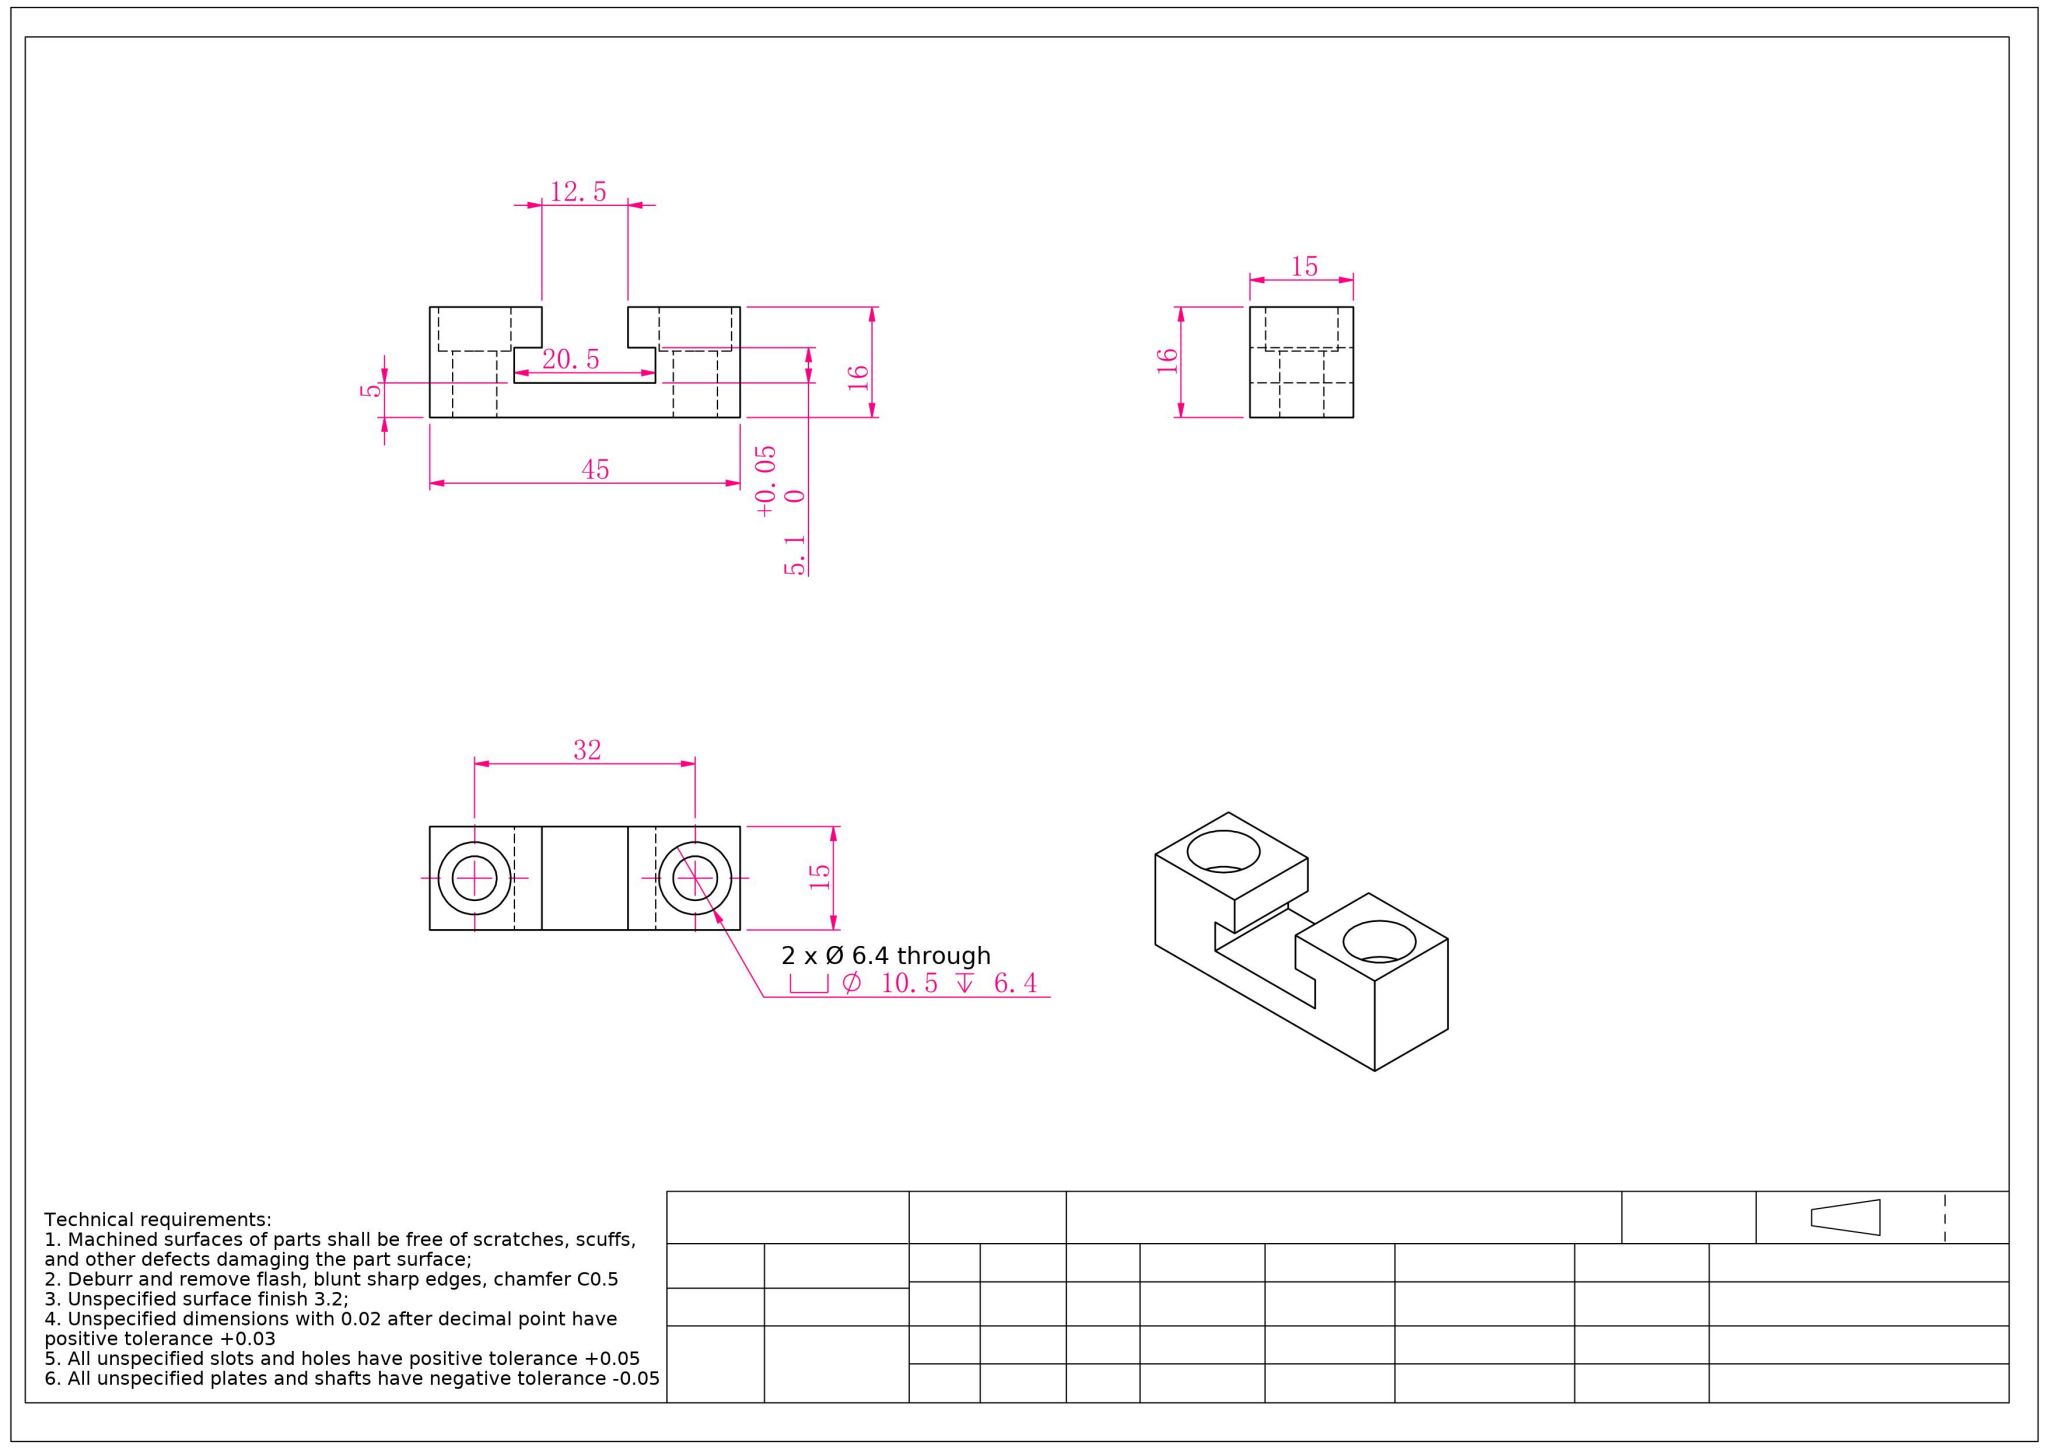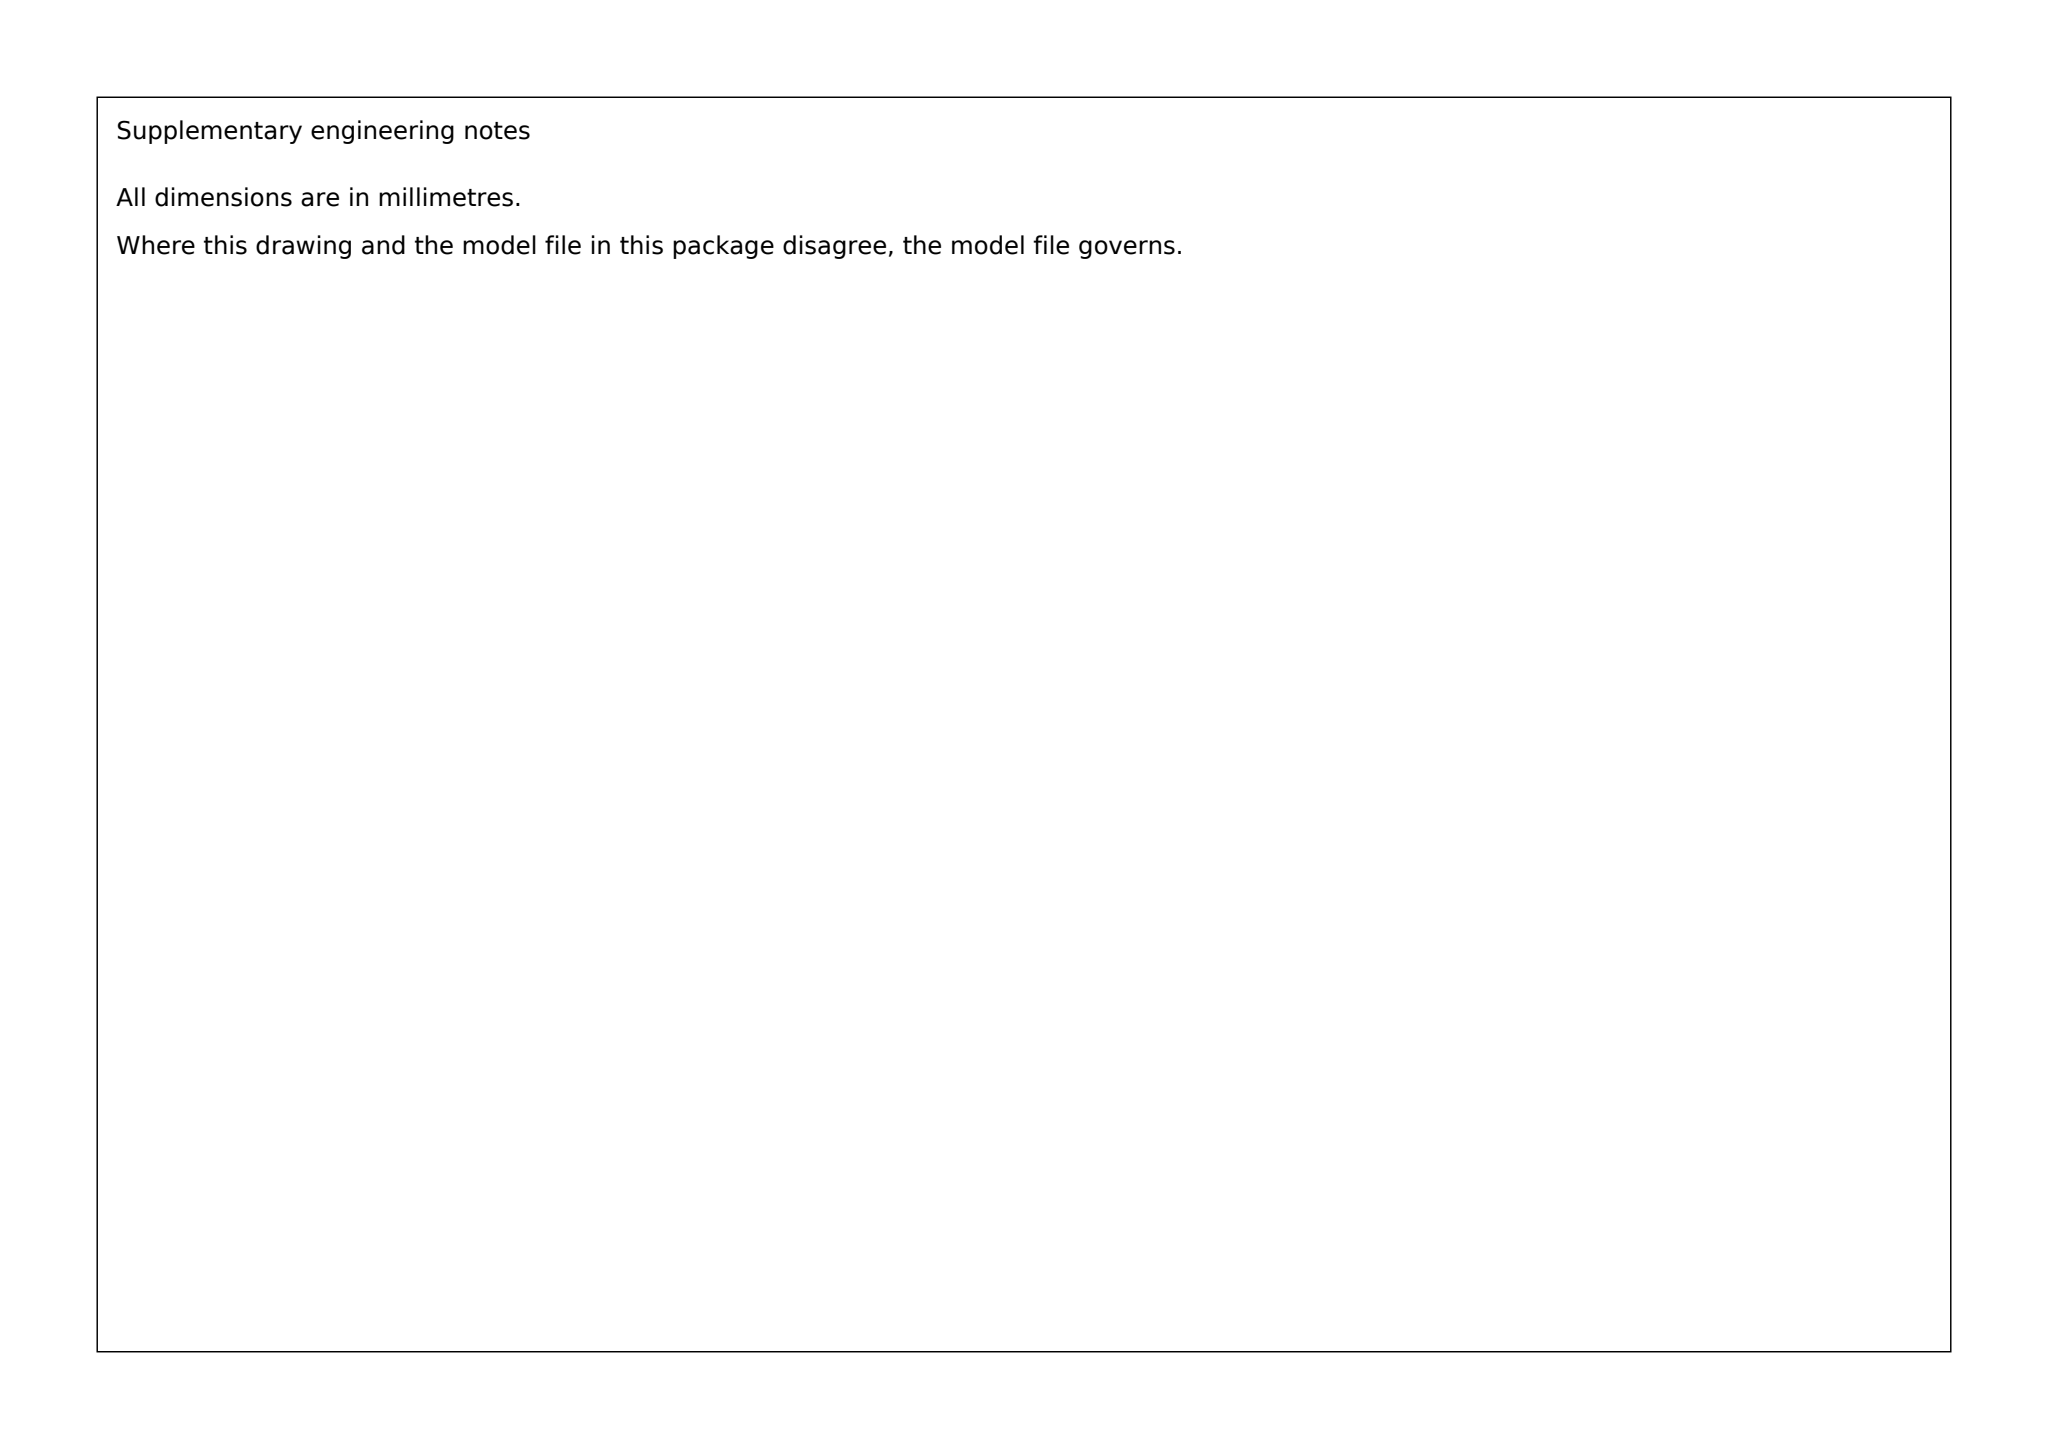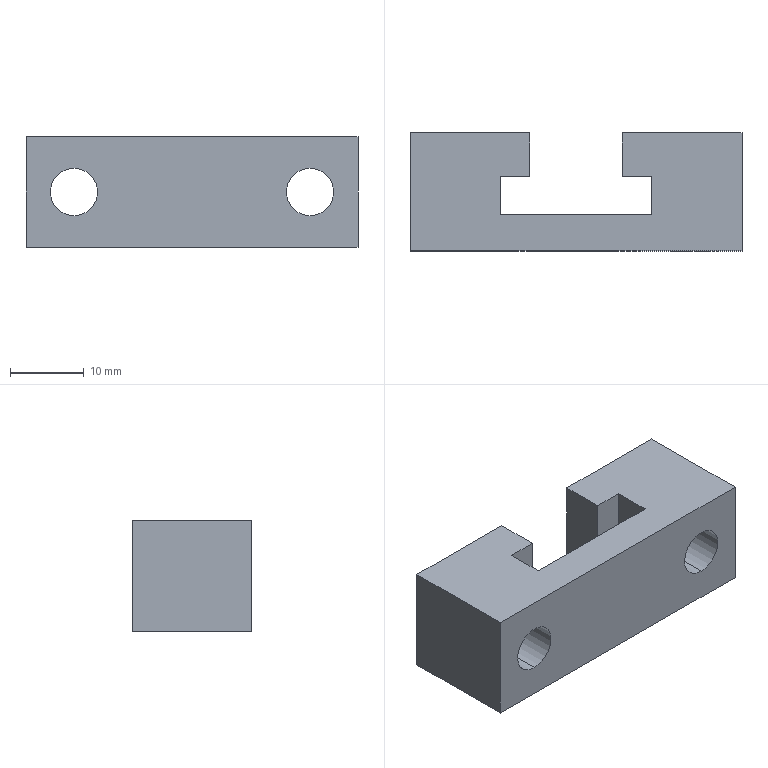Part | SolidWorks | mm | 1 solid | 24 faces | box 45 x 16 x 15 mm | volume 6399 mm3 | plane 16 | cylinder 8 | commonest cylinder face diameters 10.5 x4 6.4 x4
build123d program:
from build123d import *

# Parameters (mm, degrees)
BOSS_EXTRUDE1_DEPTH                             = 7.5
M6_HEX_SOCKET_HEAD_CAP_SCREW_CBORE1_D           = 6.4
M6_HEX_SOCKET_HEAD_CAP_SCREW_CBORE1_CBORE_D     = 10.5
M6_HEX_SOCKET_HEAD_CAP_SCREW_CBORE1_CBORE_DEPTH = 6.4


with BuildPart() as part:
    # Sketch1 → Boss-Extrude1 (new, symmetric)
    with BuildSketch(Plane.XY):
        Polygon((-22.5, 16), (-6.25, 16), (-6.25, 10.1), (-10.25, 10.1), (-10.25, 5), (10.25, 5), (10.25, 10.1), (6.25, 10.1), (6.25, 16), (22.5, 16), (22.5, 0), (-22.5, 0), align=None)
    extrude(amount=BOSS_EXTRUDE1_DEPTH, both=True)

    # M6 Hex Socket Head Cap Screw CBORE1 (through all)
    with Locations(Plane(origin=(0, 16, 0), x_dir=(1, 0, 0), z_dir=(0, 1, 0))):
        with Locations((-16, 0), (16, 0)):
            CounterBoreHole(M6_HEX_SOCKET_HEAD_CAP_SCREW_CBORE1_D / 2, M6_HEX_SOCKET_HEAD_CAP_SCREW_CBORE1_CBORE_D / 2, M6_HEX_SOCKET_HEAD_CAP_SCREW_CBORE1_CBORE_DEPTH)


solid = part.part
STEP:
#1=CARTESIAN_POINT('',(-16.,9.6,-5.25));
#2=VERTEX_POINT('',#1);
#3=CARTESIAN_POINT('',(-16.,9.6,5.25));
#4=VERTEX_POINT('',#3);
#5=CARTESIAN_POINT('',(-16.,9.6,0.));
#6=DIRECTION('',(0.,1.,0.));
#7=DIRECTION('',(0.,0.,1.));
#8=AXIS2_PLACEMENT_3D('',#5,#6,#7);
#9=CIRCLE('',#8,5.25);
#10=EDGE_CURVE('',#2,#4,#9,.T.);
#11=ORIENTED_EDGE('',*,*,#10,.F.);
#12=CARTESIAN_POINT('',(-16.,16.,-5.25));
#13=VERTEX_POINT('',#12);
#14=CARTESIAN_POINT('',(-16.,16.,-5.25));
#15=DIRECTION('',(0.,1.,0.));
#16=VECTOR('',#15,1000.);
#17=LINE('',#14,#16);
#18=EDGE_CURVE('',#2,#13,#17,.T.);
#19=ORIENTED_EDGE('',*,*,#18,.T.);
#20=CARTESIAN_POINT('',(-16.,16.,5.25));
#21=VERTEX_POINT('',#20);
#22=CARTESIAN_POINT('',(-16.,16.,0.));
#23=DIRECTION('',(0.,1.,0.));
#24=DIRECTION('',(0.,0.,1.));
#25=AXIS2_PLACEMENT_3D('',#22,#23,#24);
#26=CIRCLE('',#25,5.25);
#27=EDGE_CURVE('',#13,#21,#26,.T.);
#28=ORIENTED_EDGE('',*,*,#27,.T.);
#29=CARTESIAN_POINT('',(-16.,16.,5.25));
#30=DIRECTION('',(0.,1.,0.));
#31=VECTOR('',#30,1000.);
#32=LINE('',#29,#31);
#33=EDGE_CURVE('',#4,#21,#32,.T.);
#34=ORIENTED_EDGE('',*,*,#33,.F.);
#35=EDGE_LOOP('',(#11,#19,#28,#34));
#36=FACE_OUTER_BOUND('',#35,.T.);
#37=CARTESIAN_POINT('',(-16.,16.,0.));
#38=DIRECTION('',(0.,1.,0.));
#39=DIRECTION('',(0.,0.,1.));
#40=AXIS2_PLACEMENT_3D('',#37,#38,#39);
#41=CYLINDRICAL_SURFACE('',#40,5.25);
#42=ADVANCED_FACE('',(#36),#41,.F.);
#43=CARTESIAN_POINT('',(-16.,0.,-3.2));
#44=VERTEX_POINT('',#43);
#45=CARTESIAN_POINT('',(-16.,0.,3.2));
#46=VERTEX_POINT('',#45);
#47=CARTESIAN_POINT('',(-16.,0.,0.));
#48=DIRECTION('',(0.,1.,0.));
#49=DIRECTION('',(0.,0.,1.));
#50=AXIS2_PLACEMENT_3D('',#47,#48,#49);
#51=CIRCLE('',#50,3.2);
#52=EDGE_CURVE('',#44,#46,#51,.T.);
#53=ORIENTED_EDGE('',*,*,#52,.F.);
#54=CARTESIAN_POINT('',(-16.,9.6,-3.2));
#55=VERTEX_POINT('',#54);
#56=CARTESIAN_POINT('',(-16.,16.,-3.2));
#57=DIRECTION('',(0.,1.,0.));
#58=VECTOR('',#57,1000.);
#59=LINE('',#56,#58);
#60=EDGE_CURVE('',#44,#55,#59,.T.);
#61=ORIENTED_EDGE('',*,*,#60,.T.);
#62=CARTESIAN_POINT('',(-16.,9.6,3.2));
#63=VERTEX_POINT('',#62);
#64=CARTESIAN_POINT('',(-16.,9.6,0.));
#65=DIRECTION('',(0.,1.,0.));
#66=DIRECTION('',(0.,0.,1.));
#67=AXIS2_PLACEMENT_3D('',#64,#65,#66);
#68=CIRCLE('',#67,3.2);
#69=EDGE_CURVE('',#55,#63,#68,.T.);
#70=ORIENTED_EDGE('',*,*,#69,.T.);
#71=CARTESIAN_POINT('',(-16.,16.,3.2));
#72=DIRECTION('',(0.,1.,0.));
#73=VECTOR('',#72,1000.);
#74=LINE('',#71,#73);
#75=EDGE_CURVE('',#46,#63,#74,.T.);
#76=ORIENTED_EDGE('',*,*,#75,.F.);
#77=EDGE_LOOP('',(#53,#61,#70,#76));
#78=FACE_OUTER_BOUND('',#77,.T.);
#79=CARTESIAN_POINT('',(-16.,16.,0.));
#80=DIRECTION('',(0.,1.,0.));
#81=DIRECTION('',(0.,0.,1.));
#82=AXIS2_PLACEMENT_3D('',#79,#80,#81);
#83=CYLINDRICAL_SURFACE('',#82,3.2);
#84=ADVANCED_FACE('',(#78),#83,.F.);
#85=CARTESIAN_POINT('',(16.,9.6,-5.25));
#86=VERTEX_POINT('',#85);
#87=CARTESIAN_POINT('',(16.,9.6,5.25));
#88=VERTEX_POINT('',#87);
#89=CARTESIAN_POINT('',(16.,9.6,-0.));
#90=DIRECTION('',(0.,1.,0.));
#91=DIRECTION('',(0.,0.,1.));
#92=AXIS2_PLACEMENT_3D('',#89,#90,#91);
#93=CIRCLE('',#92,5.25);
#94=EDGE_CURVE('',#86,#88,#93,.T.);
#95=ORIENTED_EDGE('',*,*,#94,.F.);
#96=CARTESIAN_POINT('',(16.,16.,-5.25));
#97=VERTEX_POINT('',#96);
#98=CARTESIAN_POINT('',(16.,16.,-5.25));
#99=DIRECTION('',(0.,1.,0.));
#100=VECTOR('',#99,1000.);
#101=LINE('',#98,#100);
#102=EDGE_CURVE('',#86,#97,#101,.T.);
#103=ORIENTED_EDGE('',*,*,#102,.T.);
#104=CARTESIAN_POINT('',(16.,16.,5.25));
#105=VERTEX_POINT('',#104);
#106=CARTESIAN_POINT('',(16.,16.,-0.));
#107=DIRECTION('',(0.,1.,0.));
#108=DIRECTION('',(0.,0.,1.));
#109=AXIS2_PLACEMENT_3D('',#106,#107,#108);
#110=CIRCLE('',#109,5.25);
#111=EDGE_CURVE('',#97,#105,#110,.T.);
#112=ORIENTED_EDGE('',*,*,#111,.T.);
#113=CARTESIAN_POINT('',(16.,16.,5.25));
#114=DIRECTION('',(0.,1.,0.));
#115=VECTOR('',#114,1000.);
#116=LINE('',#113,#115);
#117=EDGE_CURVE('',#88,#105,#116,.T.);
#118=ORIENTED_EDGE('',*,*,#117,.F.);
#119=EDGE_LOOP('',(#95,#103,#112,#118));
#120=FACE_OUTER_BOUND('',#119,.T.);
#121=CARTESIAN_POINT('',(16.,16.,-0.));
#122=DIRECTION('',(0.,1.,0.));
#123=DIRECTION('',(0.,0.,1.));
#124=AXIS2_PLACEMENT_3D('',#121,#122,#123);
#125=CYLINDRICAL_SURFACE('',#124,5.25);
#126=ADVANCED_FACE('',(#120),#125,.F.);
#127=CARTESIAN_POINT('',(16.,0.,-3.2));
#128=VERTEX_POINT('',#127);
#129=CARTESIAN_POINT('',(16.,0.,3.2));
#130=VERTEX_POINT('',#129);
#131=CARTESIAN_POINT('',(16.,0.,-0.));
#132=DIRECTION('',(0.,1.,0.));
#133=DIRECTION('',(0.,0.,1.));
#134=AXIS2_PLACEMENT_3D('',#131,#132,#133);
#135=CIRCLE('',#134,3.2);
#136=EDGE_CURVE('',#128,#130,#135,.T.);
#137=ORIENTED_EDGE('',*,*,#136,.F.);
#138=CARTESIAN_POINT('',(16.,9.6,-3.2));
#139=VERTEX_POINT('',#138);
#140=CARTESIAN_POINT('',(16.,16.,-3.2));
#141=DIRECTION('',(0.,1.,0.));
#142=VECTOR('',#141,1000.);
#143=LINE('',#140,#142);
#144=EDGE_CURVE('',#128,#139,#143,.T.);
#145=ORIENTED_EDGE('',*,*,#144,.T.);
#146=CARTESIAN_POINT('',(16.,9.6,3.2));
#147=VERTEX_POINT('',#146);
#148=CARTESIAN_POINT('',(16.,9.6,-0.));
#149=DIRECTION('',(0.,1.,0.));
#150=DIRECTION('',(0.,0.,1.));
#151=AXIS2_PLACEMENT_3D('',#148,#149,#150);
#152=CIRCLE('',#151,3.2);
#153=EDGE_CURVE('',#139,#147,#152,.T.);
#154=ORIENTED_EDGE('',*,*,#153,.T.);
#155=CARTESIAN_POINT('',(16.,16.,3.2));
#156=DIRECTION('',(0.,1.,0.));
#157=VECTOR('',#156,1000.);
#158=LINE('',#155,#157);
#159=EDGE_CURVE('',#130,#147,#158,.T.);
#160=ORIENTED_EDGE('',*,*,#159,.F.);
#161=EDGE_LOOP('',(#137,#145,#154,#160));
#162=FACE_OUTER_BOUND('',#161,.T.);
#163=CARTESIAN_POINT('',(16.,16.,-0.));
#164=DIRECTION('',(0.,1.,0.));
#165=DIRECTION('',(0.,0.,1.));
#166=AXIS2_PLACEMENT_3D('',#163,#164,#165);
#167=CYLINDRICAL_SURFACE('',#166,3.2);
#168=ADVANCED_FACE('',(#162),#167,.F.);
#169=CARTESIAN_POINT('',(-22.5,16.,-7.5));
#170=VERTEX_POINT('',#169);
#171=CARTESIAN_POINT('',(-22.5,0.,-7.5));
#172=VERTEX_POINT('',#171);
#173=CARTESIAN_POINT('',(-22.5,16.,-7.5));
#174=DIRECTION('',(0.,-1.,0.));
#175=VECTOR('',#174,1000.);
#176=LINE('',#173,#175);
#177=EDGE_CURVE('',#170,#172,#176,.T.);
#178=ORIENTED_EDGE('',*,*,#177,.T.);
#179=CARTESIAN_POINT('',(-22.5,0.,7.5));
#180=VERTEX_POINT('',#179);
#181=CARTESIAN_POINT('',(-22.5,0.,7.5));
#182=DIRECTION('',(0.,0.,-1.));
#183=VECTOR('',#182,1000.);
#184=LINE('',#181,#183);
#185=EDGE_CURVE('',#180,#172,#184,.T.);
#186=ORIENTED_EDGE('',*,*,#185,.F.);
#187=CARTESIAN_POINT('',(-22.5,16.,7.5));
#188=VERTEX_POINT('',#187);
#189=CARTESIAN_POINT('',(-22.5,16.,7.5));
#190=DIRECTION('',(0.,-1.,0.));
#191=VECTOR('',#190,1000.);
#192=LINE('',#189,#191);
#193=EDGE_CURVE('',#188,#180,#192,.T.);
#194=ORIENTED_EDGE('',*,*,#193,.F.);
#195=CARTESIAN_POINT('',(-22.5,16.,7.5));
#196=DIRECTION('',(0.,0.,-1.));
#197=VECTOR('',#196,1000.);
#198=LINE('',#195,#197);
#199=EDGE_CURVE('',#188,#170,#198,.T.);
#200=ORIENTED_EDGE('',*,*,#199,.T.);
#201=EDGE_LOOP('',(#178,#186,#194,#200));
#202=FACE_OUTER_BOUND('',#201,.T.);
#203=CARTESIAN_POINT('',(-22.5,16.,7.5));
#204=DIRECTION('',(1.,0.,0.));
#205=DIRECTION('',(-0.,1.,0.));
#206=AXIS2_PLACEMENT_3D('',#203,#204,#205);
#207=PLANE('',#206);
#208=ADVANCED_FACE('',(#202),#207,.F.);
#209=CARTESIAN_POINT('',(-16.,0.,0.));
#210=DIRECTION('',(0.,1.,0.));
#211=DIRECTION('',(0.,0.,1.));
#212=AXIS2_PLACEMENT_3D('',#209,#210,#211);
#213=CIRCLE('',#212,3.2);
#214=EDGE_CURVE('',#46,#44,#213,.T.);
#215=ORIENTED_EDGE('',*,*,#214,.T.);
#216=ORIENTED_EDGE('',*,*,#52,.T.);
#217=EDGE_LOOP('',(#215,#216));
#218=FACE_BOUND('',#217,.T.);
#219=CARTESIAN_POINT('',(16.,0.,-0.));
#220=DIRECTION('',(0.,1.,0.));
#221=DIRECTION('',(0.,0.,1.));
#222=AXIS2_PLACEMENT_3D('',#219,#220,#221);
#223=CIRCLE('',#222,3.2);
#224=EDGE_CURVE('',#130,#128,#223,.T.);
#225=ORIENTED_EDGE('',*,*,#224,.T.);
#226=ORIENTED_EDGE('',*,*,#136,.T.);
#227=EDGE_LOOP('',(#225,#226));
#228=FACE_BOUND('',#227,.T.);
#229=CARTESIAN_POINT('',(22.5,0.,-7.5));
#230=VERTEX_POINT('',#229);
#231=CARTESIAN_POINT('',(-22.5,0.,-7.5));
#232=DIRECTION('',(1.,0.,0.));
#233=VECTOR('',#232,1000.);
#234=LINE('',#231,#233);
#235=EDGE_CURVE('',#172,#230,#234,.T.);
#236=ORIENTED_EDGE('',*,*,#235,.T.);
#237=CARTESIAN_POINT('',(22.5,0.,7.5));
#238=VERTEX_POINT('',#237);
#239=CARTESIAN_POINT('',(22.5,0.,7.5));
#240=DIRECTION('',(0.,0.,-1.));
#241=VECTOR('',#240,1000.);
#242=LINE('',#239,#241);
#243=EDGE_CURVE('',#238,#230,#242,.T.);
#244=ORIENTED_EDGE('',*,*,#243,.F.);
#245=CARTESIAN_POINT('',(-22.5,0.,7.5));
#246=DIRECTION('',(1.,0.,0.));
#247=VECTOR('',#246,1000.);
#248=LINE('',#245,#247);
#249=EDGE_CURVE('',#180,#238,#248,.T.);
#250=ORIENTED_EDGE('',*,*,#249,.F.);
#251=ORIENTED_EDGE('',*,*,#185,.T.);
#252=EDGE_LOOP('',(#236,#244,#250,#251));
#253=FACE_OUTER_BOUND('',#252,.T.);
#254=CARTESIAN_POINT('',(-22.5,0.,7.5));
#255=DIRECTION('',(0.,1.,0.));
#256=DIRECTION('',(0.,0.,1.));
#257=AXIS2_PLACEMENT_3D('',#254,#255,#256);
#258=PLANE('',#257);
#259=ADVANCED_FACE('',(#218,#228,#253),#258,.F.);
#260=CARTESIAN_POINT('',(22.5,16.,-7.5));
#261=VERTEX_POINT('',#260);
#262=CARTESIAN_POINT('',(22.5,16.,-7.5));
#263=DIRECTION('',(0.,1.,0.));
#264=VECTOR('',#263,1000.);
#265=LINE('',#262,#264);
#266=EDGE_CURVE('',#230,#261,#265,.T.);
#267=ORIENTED_EDGE('',*,*,#266,.T.);
#268=CARTESIAN_POINT('',(22.5,16.,7.5));
#269=VERTEX_POINT('',#268);
#270=CARTESIAN_POINT('',(22.5,16.,7.5));
#271=DIRECTION('',(0.,0.,-1.));
#272=VECTOR('',#271,1000.);
#273=LINE('',#270,#272);
#274=EDGE_CURVE('',#269,#261,#273,.T.);
#275=ORIENTED_EDGE('',*,*,#274,.F.);
#276=CARTESIAN_POINT('',(22.5,16.,7.5));
#277=DIRECTION('',(0.,1.,0.));
#278=VECTOR('',#277,1000.);
#279=LINE('',#276,#278);
#280=EDGE_CURVE('',#238,#269,#279,.T.);
#281=ORIENTED_EDGE('',*,*,#280,.F.);
#282=ORIENTED_EDGE('',*,*,#243,.T.);
#283=EDGE_LOOP('',(#267,#275,#281,#282));
#284=FACE_OUTER_BOUND('',#283,.T.);
#285=CARTESIAN_POINT('',(22.5,16.,7.5));
#286=DIRECTION('',(-1.,0.,0.));
#287=DIRECTION('',(-0.,-1.,0.));
#288=AXIS2_PLACEMENT_3D('',#285,#286,#287);
#289=PLANE('',#288);
#290=ADVANCED_FACE('',(#284),#289,.F.);
#291=CARTESIAN_POINT('',(16.,16.,-0.));
#292=DIRECTION('',(0.,1.,0.));
#293=DIRECTION('',(0.,0.,1.));
#294=AXIS2_PLACEMENT_3D('',#291,#292,#293);
#295=CIRCLE('',#294,5.25);
#296=EDGE_CURVE('',#105,#97,#295,.T.);
#297=ORIENTED_EDGE('',*,*,#296,.F.);
#298=ORIENTED_EDGE('',*,*,#111,.F.);
#299=EDGE_LOOP('',(#297,#298));
#300=FACE_BOUND('',#299,.T.);
#301=CARTESIAN_POINT('',(6.25,16.,-7.5));
#302=VERTEX_POINT('',#301);
#303=CARTESIAN_POINT('',(6.25,16.,-7.5));
#304=DIRECTION('',(-1.,0.,0.));
#305=VECTOR('',#304,1000.);
#306=LINE('',#303,#305);
#307=EDGE_CURVE('',#261,#302,#306,.T.);
#308=ORIENTED_EDGE('',*,*,#307,.T.);
#309=CARTESIAN_POINT('',(6.25,16.,7.5));
#310=VERTEX_POINT('',#309);
#311=CARTESIAN_POINT('',(6.25,16.,7.5));
#312=DIRECTION('',(0.,0.,-1.));
#313=VECTOR('',#312,1000.);
#314=LINE('',#311,#313);
#315=EDGE_CURVE('',#310,#302,#314,.T.);
#316=ORIENTED_EDGE('',*,*,#315,.F.);
#317=CARTESIAN_POINT('',(6.25,16.,7.5));
#318=DIRECTION('',(-1.,0.,0.));
#319=VECTOR('',#318,1000.);
#320=LINE('',#317,#319);
#321=EDGE_CURVE('',#269,#310,#320,.T.);
#322=ORIENTED_EDGE('',*,*,#321,.F.);
#323=ORIENTED_EDGE('',*,*,#274,.T.);
#324=EDGE_LOOP('',(#308,#316,#322,#323));
#325=FACE_OUTER_BOUND('',#324,.T.);
#326=CARTESIAN_POINT('',(6.25,16.,7.5));
#327=DIRECTION('',(0.,-1.,0.));
#328=DIRECTION('',(0.,0.,-1.));
#329=AXIS2_PLACEMENT_3D('',#326,#327,#328);
#330=PLANE('',#329);
#331=ADVANCED_FACE('',(#300,#325),#330,.F.);
#332=CARTESIAN_POINT('',(6.25,10.1,-7.5));
#333=VERTEX_POINT('',#332);
#334=CARTESIAN_POINT('',(6.25,16.,-7.5));
#335=DIRECTION('',(-0.,-1.,0.));
#336=VECTOR('',#335,1000.);
#337=LINE('',#334,#336);
#338=EDGE_CURVE('',#302,#333,#337,.T.);
#339=ORIENTED_EDGE('',*,*,#338,.T.);
#340=CARTESIAN_POINT('',(6.25,10.1,7.5));
#341=VERTEX_POINT('',#340);
#342=CARTESIAN_POINT('',(6.25,10.1,7.5));
#343=DIRECTION('',(0.,0.,-1.));
#344=VECTOR('',#343,1000.);
#345=LINE('',#342,#344);
#346=EDGE_CURVE('',#341,#333,#345,.T.);
#347=ORIENTED_EDGE('',*,*,#346,.F.);
#348=CARTESIAN_POINT('',(6.25,16.,7.5));
#349=DIRECTION('',(-0.,-1.,0.));
#350=VECTOR('',#349,1000.);
#351=LINE('',#348,#350);
#352=EDGE_CURVE('',#310,#341,#351,.T.);
#353=ORIENTED_EDGE('',*,*,#352,.F.);
#354=ORIENTED_EDGE('',*,*,#315,.T.);
#355=EDGE_LOOP('',(#339,#347,#353,#354));
#356=FACE_OUTER_BOUND('',#355,.T.);
#357=CARTESIAN_POINT('',(6.25,16.,7.5));
#358=DIRECTION('',(1.,-0.,0.));
#359=DIRECTION('',(0.,1.,0.));
#360=AXIS2_PLACEMENT_3D('',#357,#358,#359);
#361=PLANE('',#360);
#362=ADVANCED_FACE('',(#356),#361,.F.);
#363=CARTESIAN_POINT('',(10.25,10.1,-7.5));
#364=VERTEX_POINT('',#363);
#365=CARTESIAN_POINT('',(6.25,10.1,-7.5));
#366=DIRECTION('',(1.,0.,0.));
#367=VECTOR('',#366,1000.);
#368=LINE('',#365,#367);
#369=EDGE_CURVE('',#333,#364,#368,.T.);
#370=ORIENTED_EDGE('',*,*,#369,.T.);
#371=CARTESIAN_POINT('',(10.25,10.1,7.5));
#372=VERTEX_POINT('',#371);
#373=CARTESIAN_POINT('',(10.25,10.1,7.5));
#374=DIRECTION('',(0.,0.,-1.));
#375=VECTOR('',#374,1000.);
#376=LINE('',#373,#375);
#377=EDGE_CURVE('',#372,#364,#376,.T.);
#378=ORIENTED_EDGE('',*,*,#377,.F.);
#379=CARTESIAN_POINT('',(6.25,10.1,7.5));
#380=DIRECTION('',(1.,0.,0.));
#381=VECTOR('',#380,1000.);
#382=LINE('',#379,#381);
#383=EDGE_CURVE('',#341,#372,#382,.T.);
#384=ORIENTED_EDGE('',*,*,#383,.F.);
#385=ORIENTED_EDGE('',*,*,#346,.T.);
#386=EDGE_LOOP('',(#370,#378,#384,#385));
#387=FACE_OUTER_BOUND('',#386,.T.);
#388=CARTESIAN_POINT('',(6.25,10.1,7.5));
#389=DIRECTION('',(0.,1.,0.));
#390=DIRECTION('',(0.,0.,1.));
#391=AXIS2_PLACEMENT_3D('',#388,#389,#390);
#392=PLANE('',#391);
#393=ADVANCED_FACE('',(#387),#392,.F.);
#394=CARTESIAN_POINT('',(10.25,5.,-7.5));
#395=VERTEX_POINT('',#394);
#396=CARTESIAN_POINT('',(10.25,10.1,-7.5));
#397=DIRECTION('',(-0.,-1.,0.));
#398=VECTOR('',#397,1000.);
#399=LINE('',#396,#398);
#400=EDGE_CURVE('',#364,#395,#399,.T.);
#401=ORIENTED_EDGE('',*,*,#400,.T.);
#402=CARTESIAN_POINT('',(10.25,5.,7.5));
#403=VERTEX_POINT('',#402);
#404=CARTESIAN_POINT('',(10.25,5.,7.5));
#405=DIRECTION('',(0.,0.,-1.));
#406=VECTOR('',#405,1000.);
#407=LINE('',#404,#406);
#408=EDGE_CURVE('',#403,#395,#407,.T.);
#409=ORIENTED_EDGE('',*,*,#408,.F.);
#410=CARTESIAN_POINT('',(10.25,10.1,7.5));
#411=DIRECTION('',(-0.,-1.,0.));
#412=VECTOR('',#411,1000.);
#413=LINE('',#410,#412);
#414=EDGE_CURVE('',#372,#403,#413,.T.);
#415=ORIENTED_EDGE('',*,*,#414,.F.);
#416=ORIENTED_EDGE('',*,*,#377,.T.);
#417=EDGE_LOOP('',(#401,#409,#415,#416));
#418=FACE_OUTER_BOUND('',#417,.T.);
#419=CARTESIAN_POINT('',(10.25,10.1,7.5));
#420=DIRECTION('',(1.,-0.,0.));
#421=DIRECTION('',(0.,1.,0.));
#422=AXIS2_PLACEMENT_3D('',#419,#420,#421);
#423=PLANE('',#422);
#424=ADVANCED_FACE('',(#418),#423,.F.);
#425=CARTESIAN_POINT('',(-10.25,5.,-7.5));
#426=VERTEX_POINT('',#425);
#427=CARTESIAN_POINT('',(-10.25,5.,-7.5));
#428=DIRECTION('',(-1.,0.,0.));
#429=VECTOR('',#428,1000.);
#430=LINE('',#427,#429);
#431=EDGE_CURVE('',#395,#426,#430,.T.);
#432=ORIENTED_EDGE('',*,*,#431,.T.);
#433=CARTESIAN_POINT('',(-10.25,5.,7.5));
#434=VERTEX_POINT('',#433);
#435=CARTESIAN_POINT('',(-10.25,5.,7.5));
#436=DIRECTION('',(0.,0.,-1.));
#437=VECTOR('',#436,1000.);
#438=LINE('',#435,#437);
#439=EDGE_CURVE('',#434,#426,#438,.T.);
#440=ORIENTED_EDGE('',*,*,#439,.F.);
#441=CARTESIAN_POINT('',(-10.25,5.,7.5));
#442=DIRECTION('',(-1.,0.,0.));
#443=VECTOR('',#442,1000.);
#444=LINE('',#441,#443);
#445=EDGE_CURVE('',#403,#434,#444,.T.);
#446=ORIENTED_EDGE('',*,*,#445,.F.);
#447=ORIENTED_EDGE('',*,*,#408,.T.);
#448=EDGE_LOOP('',(#432,#440,#446,#447));
#449=FACE_OUTER_BOUND('',#448,.T.);
#450=CARTESIAN_POINT('',(-10.25,5.,7.5));
#451=DIRECTION('',(0.,-1.,0.));
#452=DIRECTION('',(0.,0.,-1.));
#453=AXIS2_PLACEMENT_3D('',#450,#451,#452);
#454=PLANE('',#453);
#455=ADVANCED_FACE('',(#449),#454,.F.);
#456=CARTESIAN_POINT('',(-10.25,10.1,-7.5));
#457=VERTEX_POINT('',#456);
#458=CARTESIAN_POINT('',(-10.25,10.1,-7.5));
#459=DIRECTION('',(-0.,1.,0.));
#460=VECTOR('',#459,1000.);
#461=LINE('',#458,#460);
#462=EDGE_CURVE('',#426,#457,#461,.T.);
#463=ORIENTED_EDGE('',*,*,#462,.T.);
#464=CARTESIAN_POINT('',(-10.25,10.1,7.5));
#465=VERTEX_POINT('',#464);
#466=CARTESIAN_POINT('',(-10.25,10.1,7.5));
#467=DIRECTION('',(0.,0.,-1.));
#468=VECTOR('',#467,1000.);
#469=LINE('',#466,#468);
#470=EDGE_CURVE('',#465,#457,#469,.T.);
#471=ORIENTED_EDGE('',*,*,#470,.F.);
#472=CARTESIAN_POINT('',(-10.25,10.1,7.5));
#473=DIRECTION('',(-0.,1.,0.));
#474=VECTOR('',#473,1000.);
#475=LINE('',#472,#474);
#476=EDGE_CURVE('',#434,#465,#475,.T.);
#477=ORIENTED_EDGE('',*,*,#476,.F.);
#478=ORIENTED_EDGE('',*,*,#439,.T.);
#479=EDGE_LOOP('',(#463,#471,#477,#478));
#480=FACE_OUTER_BOUND('',#479,.T.);
#481=CARTESIAN_POINT('',(-10.25,10.1,7.5));
#482=DIRECTION('',(-1.,-0.,0.));
#483=DIRECTION('',(0.,-1.,0.));
#484=AXIS2_PLACEMENT_3D('',#481,#482,#483);
#485=PLANE('',#484);
#486=ADVANCED_FACE('',(#480),#485,.F.);
#487=CARTESIAN_POINT('',(-6.25,10.1,-7.5));
#488=VERTEX_POINT('',#487);
#489=CARTESIAN_POINT('',(-10.25,10.1,-7.5));
#490=DIRECTION('',(1.,0.,0.));
#491=VECTOR('',#490,1000.);
#492=LINE('',#489,#491);
#493=EDGE_CURVE('',#457,#488,#492,.T.);
#494=ORIENTED_EDGE('',*,*,#493,.T.);
#495=CARTESIAN_POINT('',(-6.25,10.1,7.5));
#496=VERTEX_POINT('',#495);
#497=CARTESIAN_POINT('',(-6.25,10.1,7.5));
#498=DIRECTION('',(0.,0.,-1.));
#499=VECTOR('',#498,1000.);
#500=LINE('',#497,#499);
#501=EDGE_CURVE('',#496,#488,#500,.T.);
#502=ORIENTED_EDGE('',*,*,#501,.F.);
#503=CARTESIAN_POINT('',(-10.25,10.1,7.5));
#504=DIRECTION('',(1.,0.,0.));
#505=VECTOR('',#504,1000.);
#506=LINE('',#503,#505);
#507=EDGE_CURVE('',#465,#496,#506,.T.);
#508=ORIENTED_EDGE('',*,*,#507,.F.);
#509=ORIENTED_EDGE('',*,*,#470,.T.);
#510=EDGE_LOOP('',(#494,#502,#508,#509));
#511=FACE_OUTER_BOUND('',#510,.T.);
#512=CARTESIAN_POINT('',(-10.25,10.1,7.5));
#513=DIRECTION('',(0.,1.,0.));
#514=DIRECTION('',(0.,0.,1.));
#515=AXIS2_PLACEMENT_3D('',#512,#513,#514);
#516=PLANE('',#515);
#517=ADVANCED_FACE('',(#511),#516,.F.);
#518=CARTESIAN_POINT('',(-6.25,16.,-7.5));
#519=VERTEX_POINT('',#518);
#520=CARTESIAN_POINT('',(-6.25,16.,-7.5));
#521=DIRECTION('',(-0.,1.,0.));
#522=VECTOR('',#521,1000.);
#523=LINE('',#520,#522);
#524=EDGE_CURVE('',#488,#519,#523,.T.);
#525=ORIENTED_EDGE('',*,*,#524,.T.);
#526=CARTESIAN_POINT('',(-6.25,16.,7.5));
#527=VERTEX_POINT('',#526);
#528=CARTESIAN_POINT('',(-6.25,16.,7.5));
#529=DIRECTION('',(0.,0.,-1.));
#530=VECTOR('',#529,1000.);
#531=LINE('',#528,#530);
#532=EDGE_CURVE('',#527,#519,#531,.T.);
#533=ORIENTED_EDGE('',*,*,#532,.F.);
#534=CARTESIAN_POINT('',(-6.25,16.,7.5));
#535=DIRECTION('',(-0.,1.,0.));
#536=VECTOR('',#535,1000.);
#537=LINE('',#534,#536);
#538=EDGE_CURVE('',#496,#527,#537,.T.);
#539=ORIENTED_EDGE('',*,*,#538,.F.);
#540=ORIENTED_EDGE('',*,*,#501,.T.);
#541=EDGE_LOOP('',(#525,#533,#539,#540));
#542=FACE_OUTER_BOUND('',#541,.T.);
#543=CARTESIAN_POINT('',(-6.25,16.,7.5));
#544=DIRECTION('',(-1.,-0.,0.));
#545=DIRECTION('',(0.,-1.,0.));
#546=AXIS2_PLACEMENT_3D('',#543,#544,#545);
#547=PLANE('',#546);
#548=ADVANCED_FACE('',(#542),#547,.F.);
#549=CARTESIAN_POINT('',(-16.,16.,0.));
#550=DIRECTION('',(0.,1.,0.));
#551=DIRECTION('',(0.,0.,1.));
#552=AXIS2_PLACEMENT_3D('',#549,#550,#551);
#553=CIRCLE('',#552,5.25);
#554=EDGE_CURVE('',#21,#13,#553,.T.);
#555=ORIENTED_EDGE('',*,*,#554,.F.);
#556=ORIENTED_EDGE('',*,*,#27,.F.);
#557=EDGE_LOOP('',(#555,#556));
#558=FACE_BOUND('',#557,.T.);
#559=CARTESIAN_POINT('',(-22.5,16.,-7.5));
#560=DIRECTION('',(-1.,0.,0.));
#561=VECTOR('',#560,1000.);
#562=LINE('',#559,#561);
#563=EDGE_CURVE('',#519,#170,#562,.T.);
#564=ORIENTED_EDGE('',*,*,#563,.T.);
#565=ORIENTED_EDGE('',*,*,#199,.F.);
#566=CARTESIAN_POINT('',(-22.5,16.,7.5));
#567=DIRECTION('',(-1.,0.,0.));
#568=VECTOR('',#567,1000.);
#569=LINE('',#566,#568);
#570=EDGE_CURVE('',#527,#188,#569,.T.);
#571=ORIENTED_EDGE('',*,*,#570,.F.);
#572=ORIENTED_EDGE('',*,*,#532,.T.);
#573=EDGE_LOOP('',(#564,#565,#571,#572));
#574=FACE_OUTER_BOUND('',#573,.T.);
#575=CARTESIAN_POINT('',(-22.5,16.,7.5));
#576=DIRECTION('',(0.,-1.,0.));
#577=DIRECTION('',(0.,0.,-1.));
#578=AXIS2_PLACEMENT_3D('',#575,#576,#577);
#579=PLANE('',#578);
#580=ADVANCED_FACE('',(#558,#574),#579,.F.);
#581=ORIENTED_EDGE('',*,*,#193,.T.);
#582=ORIENTED_EDGE('',*,*,#249,.T.);
#583=ORIENTED_EDGE('',*,*,#280,.T.);
#584=ORIENTED_EDGE('',*,*,#321,.T.);
#585=ORIENTED_EDGE('',*,*,#352,.T.);
#586=ORIENTED_EDGE('',*,*,#383,.T.);
#587=ORIENTED_EDGE('',*,*,#414,.T.);
#588=ORIENTED_EDGE('',*,*,#445,.T.);
#589=ORIENTED_EDGE('',*,*,#476,.T.);
#590=ORIENTED_EDGE('',*,*,#507,.T.);
#591=ORIENTED_EDGE('',*,*,#538,.T.);
#592=ORIENTED_EDGE('',*,*,#570,.T.);
#593=EDGE_LOOP('',(#581,#582,#583,#584,#585,#586,#587,#588,#589,#590,#591,#592));
#594=FACE_OUTER_BOUND('',#593,.T.);
#595=CARTESIAN_POINT('',(0.,0.,7.5));
#596=DIRECTION('',(0.,0.,1.));
#597=DIRECTION('',(1.,0.,0.));
#598=AXIS2_PLACEMENT_3D('',#595,#596,#597);
#599=PLANE('',#598);
#600=ADVANCED_FACE('',(#594),#599,.T.);
#601=ORIENTED_EDGE('',*,*,#177,.F.);
#602=ORIENTED_EDGE('',*,*,#563,.F.);
#603=ORIENTED_EDGE('',*,*,#524,.F.);
#604=ORIENTED_EDGE('',*,*,#493,.F.);
#605=ORIENTED_EDGE('',*,*,#462,.F.);
#606=ORIENTED_EDGE('',*,*,#431,.F.);
#607=ORIENTED_EDGE('',*,*,#400,.F.);
#608=ORIENTED_EDGE('',*,*,#369,.F.);
#609=ORIENTED_EDGE('',*,*,#338,.F.);
#610=ORIENTED_EDGE('',*,*,#307,.F.);
#611=ORIENTED_EDGE('',*,*,#266,.F.);
#612=ORIENTED_EDGE('',*,*,#235,.F.);
#613=EDGE_LOOP('',(#601,#602,#603,#604,#605,#606,#607,#608,#609,#610,#611,#612));
#614=FACE_OUTER_BOUND('',#613,.T.);
#615=CARTESIAN_POINT('',(0.,0.,-7.5));
#616=DIRECTION('',(0.,0.,1.));
#617=DIRECTION('',(1.,0.,0.));
#618=AXIS2_PLACEMENT_3D('',#615,#616,#617);
#619=PLANE('',#618);
#620=ADVANCED_FACE('',(#614),#619,.F.);
#621=ORIENTED_EDGE('',*,*,#144,.F.);
#622=ORIENTED_EDGE('',*,*,#224,.F.);
#623=ORIENTED_EDGE('',*,*,#159,.T.);
#624=CARTESIAN_POINT('',(16.,9.6,-0.));
#625=DIRECTION('',(0.,1.,0.));
#626=DIRECTION('',(0.,0.,1.));
#627=AXIS2_PLACEMENT_3D('',#624,#625,#626);
#628=CIRCLE('',#627,3.2);
#629=EDGE_CURVE('',#147,#139,#628,.T.);
#630=ORIENTED_EDGE('',*,*,#629,.T.);
#631=EDGE_LOOP('',(#621,#622,#623,#630));
#632=FACE_OUTER_BOUND('',#631,.T.);
#633=CARTESIAN_POINT('',(16.,16.,-0.));
#634=DIRECTION('',(0.,1.,0.));
#635=DIRECTION('',(0.,0.,1.));
#636=AXIS2_PLACEMENT_3D('',#633,#634,#635);
#637=CYLINDRICAL_SURFACE('',#636,3.2);
#638=ADVANCED_FACE('',(#632),#637,.F.);
#639=ORIENTED_EDGE('',*,*,#629,.F.);
#640=ORIENTED_EDGE('',*,*,#153,.F.);
#641=EDGE_LOOP('',(#639,#640));
#642=FACE_BOUND('',#641,.T.);
#643=CARTESIAN_POINT('',(16.,9.6,-0.));
#644=DIRECTION('',(0.,1.,0.));
#645=DIRECTION('',(0.,0.,1.));
#646=AXIS2_PLACEMENT_3D('',#643,#644,#645);
#647=CIRCLE('',#646,5.25);
#648=EDGE_CURVE('',#88,#86,#647,.T.);
#649=ORIENTED_EDGE('',*,*,#648,.T.);
#650=ORIENTED_EDGE('',*,*,#94,.T.);
#651=EDGE_LOOP('',(#649,#650));
#652=FACE_OUTER_BOUND('',#651,.T.);
#653=CARTESIAN_POINT('',(19.2,9.6,-0.));
#654=DIRECTION('',(0.,-1.,0.));
#655=DIRECTION('',(0.,0.,-1.));
#656=AXIS2_PLACEMENT_3D('',#653,#654,#655);
#657=PLANE('',#656);
#658=ADVANCED_FACE('',(#642,#652),#657,.F.);
#659=ORIENTED_EDGE('',*,*,#102,.F.);
#660=ORIENTED_EDGE('',*,*,#648,.F.);
#661=ORIENTED_EDGE('',*,*,#117,.T.);
#662=ORIENTED_EDGE('',*,*,#296,.T.);
#663=EDGE_LOOP('',(#659,#660,#661,#662));
#664=FACE_OUTER_BOUND('',#663,.T.);
#665=CARTESIAN_POINT('',(16.,16.,-0.));
#666=DIRECTION('',(0.,1.,0.));
#667=DIRECTION('',(0.,0.,1.));
#668=AXIS2_PLACEMENT_3D('',#665,#666,#667);
#669=CYLINDRICAL_SURFACE('',#668,5.25);
#670=ADVANCED_FACE('',(#664),#669,.F.);
#671=ORIENTED_EDGE('',*,*,#60,.F.);
#672=ORIENTED_EDGE('',*,*,#214,.F.);
#673=ORIENTED_EDGE('',*,*,#75,.T.);
#674=CARTESIAN_POINT('',(-16.,9.6,0.));
#675=DIRECTION('',(0.,1.,0.));
#676=DIRECTION('',(0.,0.,1.));
#677=AXIS2_PLACEMENT_3D('',#674,#675,#676);
#678=CIRCLE('',#677,3.2);
#679=EDGE_CURVE('',#63,#55,#678,.T.);
#680=ORIENTED_EDGE('',*,*,#679,.T.);
#681=EDGE_LOOP('',(#671,#672,#673,#680));
#682=FACE_OUTER_BOUND('',#681,.T.);
#683=CARTESIAN_POINT('',(-16.,16.,0.));
#684=DIRECTION('',(0.,1.,0.));
#685=DIRECTION('',(0.,0.,1.));
#686=AXIS2_PLACEMENT_3D('',#683,#684,#685);
#687=CYLINDRICAL_SURFACE('',#686,3.2);
#688=ADVANCED_FACE('',(#682),#687,.F.);
#689=ORIENTED_EDGE('',*,*,#679,.F.);
#690=ORIENTED_EDGE('',*,*,#69,.F.);
#691=EDGE_LOOP('',(#689,#690));
#692=FACE_BOUND('',#691,.T.);
#693=CARTESIAN_POINT('',(-16.,9.6,0.));
#694=DIRECTION('',(0.,1.,0.));
#695=DIRECTION('',(0.,0.,1.));
#696=AXIS2_PLACEMENT_3D('',#693,#694,#695);
#697=CIRCLE('',#696,5.25);
#698=EDGE_CURVE('',#4,#2,#697,.T.);
#699=ORIENTED_EDGE('',*,*,#698,.T.);
#700=ORIENTED_EDGE('',*,*,#10,.T.);
#701=EDGE_LOOP('',(#699,#700));
#702=FACE_OUTER_BOUND('',#701,.T.);
#703=CARTESIAN_POINT('',(-12.8,9.6,0.));
#704=DIRECTION('',(0.,-1.,0.));
#705=DIRECTION('',(0.,0.,-1.));
#706=AXIS2_PLACEMENT_3D('',#703,#704,#705);
#707=PLANE('',#706);
#708=ADVANCED_FACE('',(#692,#702),#707,.F.);
#709=ORIENTED_EDGE('',*,*,#18,.F.);
#710=ORIENTED_EDGE('',*,*,#698,.F.);
#711=ORIENTED_EDGE('',*,*,#33,.T.);
#712=ORIENTED_EDGE('',*,*,#554,.T.);
#713=EDGE_LOOP('',(#709,#710,#711,#712));
#714=FACE_OUTER_BOUND('',#713,.T.);
#715=CARTESIAN_POINT('',(-16.,16.,0.));
#716=DIRECTION('',(0.,1.,0.));
#717=DIRECTION('',(0.,0.,1.));
#718=AXIS2_PLACEMENT_3D('',#715,#716,#717);
#719=CYLINDRICAL_SURFACE('',#718,5.25);
#720=ADVANCED_FACE('',(#714),#719,.F.);
#721=CLOSED_SHELL('',(#42,#84,#126,#168,#208,#259,#290,#331,#362,#393,#424,#455,#486,#517,#548,#580,#600,#620,#638,#658,#670,#688,#708,#720));
#722=MANIFOLD_SOLID_BREP('',#721);
#723=CARTESIAN_POINT('',(0.,0.,0.));
#724=DIRECTION('',(0.,0.,1.));
#725=DIRECTION('',(1.,0.,0.));
#726=AXIS2_PLACEMENT_3D('',#723,#724,#725);
#727=(LENGTH_UNIT()NAMED_UNIT(*)SI_UNIT(.MILLI.,.METRE.));
#728=UNCERTAINTY_MEASURE_WITH_UNIT(LENGTH_MEASURE(0.00001),#727,'','');
#729=(NAMED_UNIT(*)PLANE_ANGLE_UNIT()SI_UNIT($,.RADIAN.));
#730=(NAMED_UNIT(*)SI_UNIT($,.STERADIAN.)SOLID_ANGLE_UNIT());
#731=(GEOMETRIC_REPRESENTATION_CONTEXT(3)GLOBAL_UNCERTAINTY_ASSIGNED_CONTEXT((#728))GLOBAL_UNIT_ASSIGNED_CONTEXT((#727,#729,#730))REPRESENTATION_CONTEXT('',''));
#732=ADVANCED_BREP_SHAPE_REPRESENTATION('',(#722,#726),#731);